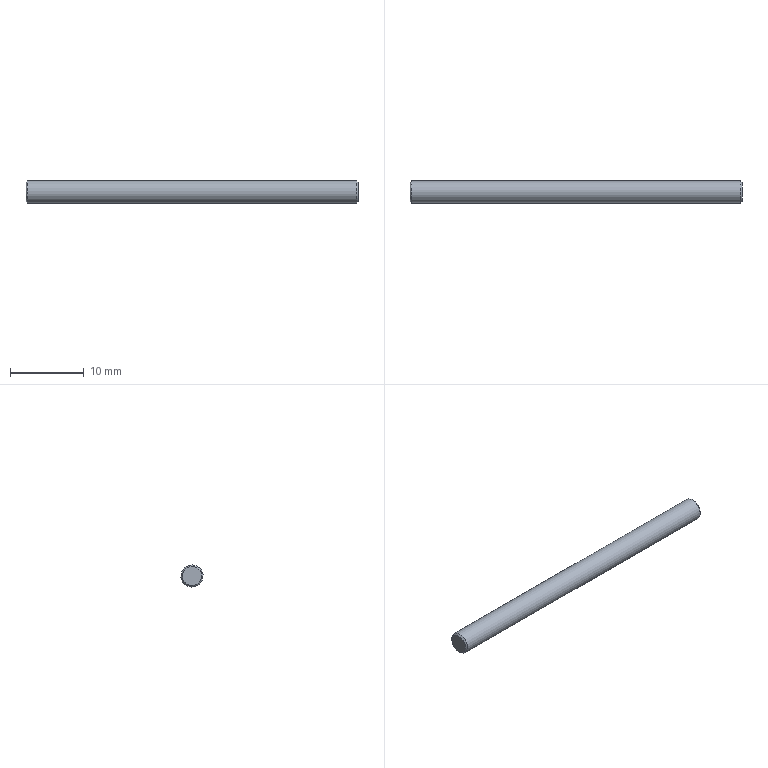Component | NX | GB120-3X45_2 | 1 solid | 5 faces | box 45 x 3 x 3 mm | volume 318 mm3 | plane 2 | cone 2 | cylinder 1 | commonest cylinder face diameters 3 x1
STEP:
#1=CARTESIAN_POINT('',(0.,0.,0.));
#2=DIRECTION('',(0.,0.,1.));
#3=DIRECTION('',(1.,0.,0.));
#4=AXIS2_PLACEMENT_3D('',#1,#2,#3);
#5=CARTESIAN_POINT('',(36.8,10.886,53.073));
#6=VERTEX_POINT('',#5);
#7=CARTESIAN_POINT('',(36.8,9.5,52.5));
#8=DIRECTION('',(-1.,0.,0.));
#9=DIRECTION('',(0.,0.9242,0.3818));
#10=AXIS2_PLACEMENT_3D('',#7,#8,#9);
#11=CIRCLE('',#10,1.5);
#12=CARTESIAN_POINT('',(37.,9.5,52.5));
#13=DIRECTION('',(-1.,0.,0.));
#14=DIRECTION('',(0.,-0.9242,-0.3818));
#15=AXIS2_PLACEMENT_3D('',#12,#13,#14);
#16=CYLINDRICAL_SURFACE('',#15,1.5);
#17=CARTESIAN_POINT('',(3.142,0.2));
#18=DIRECTION('',(1.,0.));
#19=VECTOR('',#18,1.);
#20=LINE('',#17,#19);
#21=(GEOMETRIC_REPRESENTATION_CONTEXT(2)PARAMETRIC_REPRESENTATION_CONTEXT()REPRESENTATION_CONTEXT('',''));
#22=DEFINITIONAL_REPRESENTATION('',(#20),#21);
#23=PCURVE('',#16,#22);
#24=CARTESIAN_POINT('',(37.,9.5,52.5));
#25=DIRECTION('',(-1.,0.,0.));
#26=DIRECTION('',(0.,-0.9242,-0.3818));
#27=AXIS2_PLACEMENT_3D('',#24,#25,#26);
#28=CONICAL_SURFACE('',#27,1.3,0.7854);
#29=CARTESIAN_POINT('',(3.142,0.2));
#30=DIRECTION('',(1.,0.));
#31=VECTOR('',#30,1.);
#32=LINE('',#29,#31);
#33=(GEOMETRIC_REPRESENTATION_CONTEXT(2)PARAMETRIC_REPRESENTATION_CONTEXT()REPRESENTATION_CONTEXT('',''));
#34=DEFINITIONAL_REPRESENTATION('',(#32),#33);
#35=PCURVE('',#28,#34);
#36=SURFACE_CURVE('',#11,(#23,#35),.PCURVE_S1.);
#37=EDGE_CURVE('',#6,#6,#36,.T.);
#38=ORIENTED_EDGE('',*,*,#37,.T.);
#39=CARTESIAN_POINT('',(-7.8,10.886,53.073));
#40=VERTEX_POINT('',#39);
#41=CARTESIAN_POINT('',(36.8,10.886,53.073));
#42=CARTESIAN_POINT('',(-7.8,10.886,53.073));
#43=B_SPLINE_CURVE_WITH_KNOTS('',1,(#41,#42),.UNSPECIFIED.,.F.,.F.,(2,2),(0.2,44.8),.PIECEWISE_BEZIER_KNOTS.);
#44=CARTESIAN_POINT('',(9.425,0.));
#45=DIRECTION('',(0.,1.));
#46=VECTOR('',#45,1.);
#47=LINE('',#44,#46);
#48=(GEOMETRIC_REPRESENTATION_CONTEXT(2)PARAMETRIC_REPRESENTATION_CONTEXT()REPRESENTATION_CONTEXT('',''));
#49=DEFINITIONAL_REPRESENTATION('',(#47),#48);
#50=PCURVE('',#16,#49);
#51=CARTESIAN_POINT('',(3.142,0.));
#52=DIRECTION('',(0.,1.));
#53=VECTOR('',#52,1.);
#54=LINE('',#51,#53);
#55=(GEOMETRIC_REPRESENTATION_CONTEXT(2)PARAMETRIC_REPRESENTATION_CONTEXT()REPRESENTATION_CONTEXT('',''));
#56=DEFINITIONAL_REPRESENTATION('',(#54),#55);
#57=PCURVE('',#16,#56);
#58=SEAM_CURVE('',#43,(#50,#57),.PCURVE_S1.);
#59=EDGE_CURVE('',#6,#40,#58,.T.);
#60=ORIENTED_EDGE('',*,*,#59,.T.);
#61=CARTESIAN_POINT('',(-7.8,9.5,52.5));
#62=DIRECTION('',(1.,0.,0.));
#63=DIRECTION('',(0.,0.9242,0.3818));
#64=AXIS2_PLACEMENT_3D('',#61,#62,#63);
#65=CIRCLE('',#64,1.5);
#66=CARTESIAN_POINT('',(9.425,44.8));
#67=DIRECTION('',(-1.,0.));
#68=VECTOR('',#67,1.);
#69=LINE('',#66,#68);
#70=(GEOMETRIC_REPRESENTATION_CONTEXT(2)PARAMETRIC_REPRESENTATION_CONTEXT()REPRESENTATION_CONTEXT('',''));
#71=DEFINITIONAL_REPRESENTATION('',(#69),#70);
#72=PCURVE('',#16,#71);
#73=CARTESIAN_POINT('',(-7.8,9.5,52.5));
#74=DIRECTION('',(1.,0.,0.));
#75=DIRECTION('',(0.,0.9242,0.3818));
#76=AXIS2_PLACEMENT_3D('',#73,#74,#75);
#77=CONICAL_SURFACE('',#76,1.5,0.7854);
#78=CARTESIAN_POINT('',(0.,0.));
#79=DIRECTION('',(1.,0.));
#80=VECTOR('',#79,1.);
#81=LINE('',#78,#80);
#82=(GEOMETRIC_REPRESENTATION_CONTEXT(2)PARAMETRIC_REPRESENTATION_CONTEXT()REPRESENTATION_CONTEXT('',''));
#83=DEFINITIONAL_REPRESENTATION('',(#81),#82);
#84=PCURVE('',#77,#83);
#85=SURFACE_CURVE('',#65,(#72,#84),.PCURVE_S1.);
#86=EDGE_CURVE('',#40,#40,#85,.T.);
#87=ORIENTED_EDGE('',*,*,#86,.T.);
#88=ORIENTED_EDGE('',*,*,#59,.F.);
#89=EDGE_LOOP('',(#38,#60,#87,#88));
#90=FACE_BOUND('',#89,.T.);
#91=ADVANCED_FACE('',(#90),#16,.T.);
#92=CARTESIAN_POINT('',(37.,10.701,52.996));
#93=VERTEX_POINT('',#92);
#94=CARTESIAN_POINT('',(37.,9.5,52.5));
#95=DIRECTION('',(1.,0.,0.));
#96=DIRECTION('',(0.,0.9242,0.3818));
#97=AXIS2_PLACEMENT_3D('',#94,#95,#96);
#98=CIRCLE('',#97,1.3);
#99=CARTESIAN_POINT('',(37.,9.5,52.5));
#100=DIRECTION('',(1.,0.,0.));
#101=DIRECTION('',(0.,0.9242,0.3818));
#102=AXIS2_PLACEMENT_3D('',#99,#100,#101);
#103=PLANE('',#102);
#104=CARTESIAN_POINT('',(0.,0.));
#105=DIRECTION('',(1.,0.));
#106=AXIS2_PLACEMENT_2D('',#104,#105);
#107=CIRCLE('',#106,1.3);
#108=(GEOMETRIC_REPRESENTATION_CONTEXT(2)PARAMETRIC_REPRESENTATION_CONTEXT()REPRESENTATION_CONTEXT('',''));
#109=DEFINITIONAL_REPRESENTATION('',(#107),#108);
#110=PCURVE('',#103,#109);
#111=CARTESIAN_POINT('',(9.425,0.));
#112=DIRECTION('',(-1.,0.));
#113=VECTOR('',#112,1.);
#114=LINE('',#111,#113);
#115=(GEOMETRIC_REPRESENTATION_CONTEXT(2)PARAMETRIC_REPRESENTATION_CONTEXT()REPRESENTATION_CONTEXT('',''));
#116=DEFINITIONAL_REPRESENTATION('',(#114),#115);
#117=PCURVE('',#28,#116);
#118=SURFACE_CURVE('',#98,(#110,#117),.PCURVE_S1.);
#119=EDGE_CURVE('',#93,#93,#118,.T.);
#120=ORIENTED_EDGE('',*,*,#119,.T.);
#121=EDGE_LOOP('',(#120));
#122=FACE_BOUND('',#121,.T.);
#123=ADVANCED_FACE('',(#122),#103,.T.);
#124=CARTESIAN_POINT('',(-8.,10.701,52.996));
#125=VERTEX_POINT('',#124);
#126=CARTESIAN_POINT('',(-8.,9.5,52.5));
#127=DIRECTION('',(-1.,0.,0.));
#128=DIRECTION('',(0.,0.9242,0.3818));
#129=AXIS2_PLACEMENT_3D('',#126,#127,#128);
#130=CIRCLE('',#129,1.3);
#131=CARTESIAN_POINT('',(-8.,9.5,52.5));
#132=DIRECTION('',(1.,0.,0.));
#133=DIRECTION('',(0.,0.9242,0.3818));
#134=AXIS2_PLACEMENT_3D('',#131,#132,#133);
#135=PLANE('',#134);
#136=CARTESIAN_POINT('',(1.3,0.));
#137=CARTESIAN_POINT('',(1.3,-2.252));
#138=CARTESIAN_POINT('',(-0.65,-1.126));
#139=CARTESIAN_POINT('',(-2.6,-0.));
#140=CARTESIAN_POINT('',(-0.65,1.126));
#141=CARTESIAN_POINT('',(1.3,2.252));
#142=CARTESIAN_POINT('',(1.3,0.));
#143=(BOUNDED_CURVE()B_SPLINE_CURVE(2,(#136,#137,#138,#139,#140,#141,#142),.UNSPECIFIED.,.T.,.F.)B_SPLINE_CURVE_WITH_KNOTS((1,2,2,2,2,1),(-2.094,0.,2.094,4.189,6.283,8.378),.UNSPECIFIED.)CURVE()GEOMETRIC_REPRESENTATION_ITEM()RATIONAL_B_SPLINE_CURVE((1.,0.5,1.,0.5,1.,0.5,1.))REPRESENTATION_ITEM(''));
#144=(GEOMETRIC_REPRESENTATION_CONTEXT(2)PARAMETRIC_REPRESENTATION_CONTEXT()REPRESENTATION_CONTEXT('',''));
#145=DEFINITIONAL_REPRESENTATION('',(#143),#144);
#146=PCURVE('',#135,#145);
#147=CARTESIAN_POINT('',(6.283,-0.2));
#148=DIRECTION('',(-1.,0.));
#149=VECTOR('',#148,1.);
#150=LINE('',#147,#149);
#151=(GEOMETRIC_REPRESENTATION_CONTEXT(2)PARAMETRIC_REPRESENTATION_CONTEXT()REPRESENTATION_CONTEXT('',''));
#152=DEFINITIONAL_REPRESENTATION('',(#150),#151);
#153=PCURVE('',#77,#152);
#154=SURFACE_CURVE('',#130,(#146,#153),.PCURVE_S1.);
#155=EDGE_CURVE('',#125,#125,#154,.T.);
#156=ORIENTED_EDGE('',*,*,#155,.T.);
#157=EDGE_LOOP('',(#156));
#158=FACE_BOUND('',#157,.T.);
#159=ADVANCED_FACE('',(#158),#135,.F.);
#160=ORIENTED_EDGE('',*,*,#37,.F.);
#161=CARTESIAN_POINT('',(37.,10.701,52.996));
#162=CARTESIAN_POINT('',(36.8,10.886,53.073));
#163=B_SPLINE_CURVE_WITH_KNOTS('',1,(#161,#162),.UNSPECIFIED.,.F.,.F.,(2,2),(0.,0.2828),.PIECEWISE_BEZIER_KNOTS.);
#164=CARTESIAN_POINT('',(3.142,0.));
#165=DIRECTION('',(0.,1.));
#166=VECTOR('',#165,1.);
#167=LINE('',#164,#166);
#168=(GEOMETRIC_REPRESENTATION_CONTEXT(2)PARAMETRIC_REPRESENTATION_CONTEXT()REPRESENTATION_CONTEXT('',''));
#169=DEFINITIONAL_REPRESENTATION('',(#167),#168);
#170=PCURVE('',#28,#169);
#171=CARTESIAN_POINT('',(9.425,0.));
#172=DIRECTION('',(0.,1.));
#173=VECTOR('',#172,1.);
#174=LINE('',#171,#173);
#175=(GEOMETRIC_REPRESENTATION_CONTEXT(2)PARAMETRIC_REPRESENTATION_CONTEXT()REPRESENTATION_CONTEXT('',''));
#176=DEFINITIONAL_REPRESENTATION('',(#174),#175);
#177=PCURVE('',#28,#176);
#178=SEAM_CURVE('',#163,(#170,#177),.PCURVE_S1.);
#179=EDGE_CURVE('',#93,#6,#178,.T.);
#180=ORIENTED_EDGE('',*,*,#179,.F.);
#181=ORIENTED_EDGE('',*,*,#119,.F.);
#182=ORIENTED_EDGE('',*,*,#179,.T.);
#183=EDGE_LOOP('',(#160,#180,#181,#182));
#184=FACE_BOUND('',#183,.T.);
#185=ADVANCED_FACE('',(#184),#28,.T.);
#186=ORIENTED_EDGE('',*,*,#155,.F.);
#187=CARTESIAN_POINT('',(-8.,10.701,52.996));
#188=CARTESIAN_POINT('',(-7.8,10.886,53.073));
#189=B_SPLINE_CURVE_WITH_KNOTS('',1,(#187,#188),.UNSPECIFIED.,.F.,.F.,(2,2),(-0.2828,0.),.PIECEWISE_BEZIER_KNOTS.);
#190=CARTESIAN_POINT('',(6.283,0.));
#191=DIRECTION('',(0.,1.));
#192=VECTOR('',#191,1.);
#193=LINE('',#190,#192);
#194=(GEOMETRIC_REPRESENTATION_CONTEXT(2)PARAMETRIC_REPRESENTATION_CONTEXT()REPRESENTATION_CONTEXT('',''));
#195=DEFINITIONAL_REPRESENTATION('',(#193),#194);
#196=PCURVE('',#77,#195);
#197=CARTESIAN_POINT('',(0.,0.));
#198=DIRECTION('',(0.,1.));
#199=VECTOR('',#198,1.);
#200=LINE('',#197,#199);
#201=(GEOMETRIC_REPRESENTATION_CONTEXT(2)PARAMETRIC_REPRESENTATION_CONTEXT()REPRESENTATION_CONTEXT('',''));
#202=DEFINITIONAL_REPRESENTATION('',(#200),#201);
#203=PCURVE('',#77,#202);
#204=SEAM_CURVE('',#189,(#196,#203),.PCURVE_S1.);
#205=EDGE_CURVE('',#125,#40,#204,.T.);
#206=ORIENTED_EDGE('',*,*,#205,.T.);
#207=ORIENTED_EDGE('',*,*,#86,.F.);
#208=ORIENTED_EDGE('',*,*,#205,.F.);
#209=EDGE_LOOP('',(#186,#206,#207,#208));
#210=FACE_BOUND('',#209,.T.);
#211=ADVANCED_FACE('',(#210),#77,.T.);
#212=CLOSED_SHELL('',(#91,#123,#159,#185,#211));
#213=MANIFOLD_SOLID_BREP('',#212);
#214=(LENGTH_UNIT()NAMED_UNIT(*)SI_UNIT(.MILLI.,.METRE.));
#215=UNCERTAINTY_MEASURE_WITH_UNIT(LENGTH_MEASURE(0.00001),#214,'','');
#216=(NAMED_UNIT(*)PLANE_ANGLE_UNIT()SI_UNIT($,.RADIAN.));
#217=(NAMED_UNIT(*)SI_UNIT($,.STERADIAN.)SOLID_ANGLE_UNIT());
#218=(GEOMETRIC_REPRESENTATION_CONTEXT(3)GLOBAL_UNCERTAINTY_ASSIGNED_CONTEXT((#215))GLOBAL_UNIT_ASSIGNED_CONTEXT((#214,#216,#217))REPRESENTATION_CONTEXT('',''));
#219=ADVANCED_BREP_SHAPE_REPRESENTATION('',(#4,#213),#218);